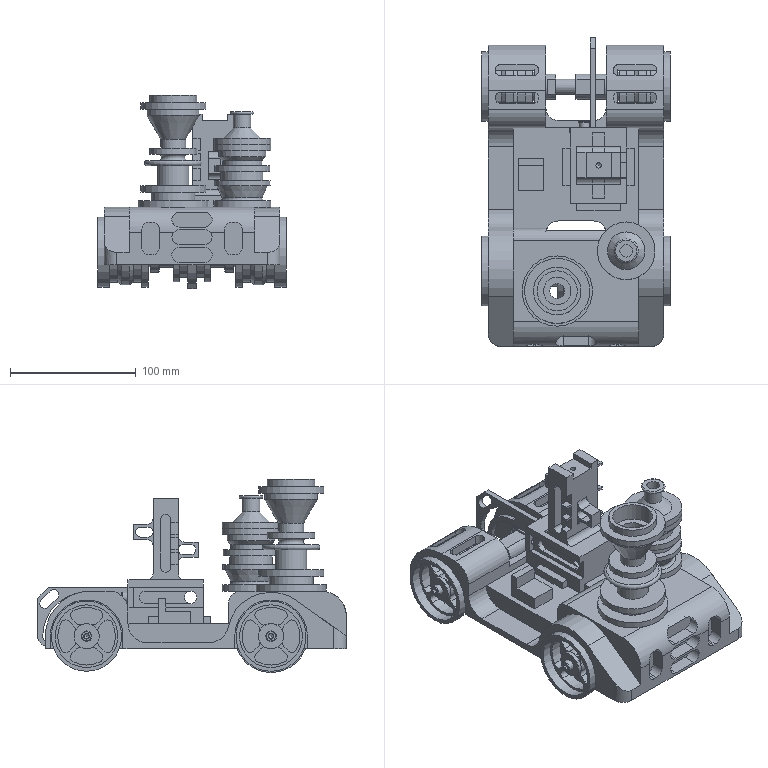Assembly | NX | mm | 29 component files | 81 solids | 972 faces | box 150 x 246 x 154 mm | volume 917936 mm3 | plane 477 | cylinder 340 | cone 83 | sphere 48 | torus 24 | commonest cylinder face diameters 8 x78 20 x49 46 x20 12 x18 28 x13 4.826 x12 16 x12 10 x10
Bill of materials:
GB-T70.1-2000,M5x10 | 6 |  | Hexagon Socket Head Cap Screw, GB-T 70.1-2000,M5x10
unnamed part 1 | 4 |  | Flat annular disc (washer-like ring) with a single concentric round through-hole; plain cylindrical outer edge.
unnamed part 2 | 1 |  | Symmetric stepped axisymmetric shaft with a central cluster of three raised flanges (tallest in the middle) flanked by stepped shoulders and long plain end journals; small axial hole at the shaft end.
unnamed part 3 | 4 |  | Spool- or rim-like axisymmetric hollow body: cylinder with raised end flanges and a raised central band with tapered edges; open end shows an inner hub with central bore connected to the rim by three curved spokes/webs.
GB-T276_60000-1994,61804 | 4 |  | Annular assembly that looks like an open radial ball bearing. It has a plain cylindrical outer ring, a concentric inner ring with a through bore, and a single row of spherical balls in the annular gap between the rings. No cage, shields or seals are visible.
unnamed part 4 | 1 |  | Axisymmetric flanged nozzle-like body: wide flat flange disc, a conical section rising to a narrow cylindrical neck with rounded bead lip at top, and a stepped cylindrical spigot below the flange; central through-bore.
unnamed part 5 | 3 |  | Plain thick-walled cylindrical tube/sleeve with a concentric through-bore and flat square ends.
unnamed part 6 | 1 |  | Stepped cylindrical shaft with several diameter changes, a narrow raised collar, a reduced neck in the middle, and flat milled faces on two of the larger sections; small axial hole at one end.
unnamed part 7 | 1 |  | Prismatic block-type body: rectangular base with side grooves/steps and a long slot, supporting a narrower vertical column with a top notch, a small top hole, side lugs with obround slots, and a row of thin horizontal fins/ribs along one side.
unnamed part 8 | 1 |  | Axisymmetric stacked-flange body: several disc flanges separated by necks, a large cup/counterbore at the top, a flared conical section with filleted root near the bottom, and a small cylindrical pin projecting from the bottom.
unnamed part 9 | 1 |  | Plate-like saddle/clamp body with two parallel half-round arched channels across its width, a flat central deck with small raised blocks and ribs, several obround slots in the arches and end wall, a large round hole with a flat (D-shaped) and small holes.
unnamed part 10 | 1 |  | Axisymmetric multi-stage body with a central through-bore: top cylindrical rim with flange, a converging funnel cone, narrow neck, a flange and rounded bead ring separated by a filleted groove, a cylindrical stem, and two lower flanges with a short bottom spigot.
unnamed part 11 | 1 |  | L-shaped flat bracket of uniform thickness: short leg with an obround slot, long arm ending in a curved hook-like lobe containing a long arcuate slot and an angled obround slot, with a chamfered corner.
Mates:
1. fix | car_body 1 component
2. concentric | support_block 1 arc | car_body 1 edge
3. concentric | lamp_body 1 edge | car_body 1 edge
4. concentric | lamp_socket 1 edge | lamp_body 1 edge
5. concentric | column 1 edge | car_body 1 edge
6. touch align | rear_axle 1 face | car_body 1 face
7. center | rear_axle 1 face | rear_axle 1 face | car_body 1 face | car_body 1 face
8. touch align | front_axle 1 face | car_body 1 face
9. center | front_axle 1 face | front_axle 1 face | car_body 1 face | car_body 1 face
10. concentric | GB-T276_60000-1994_61804 4 edge | car_body 1 edge
11. bond | car_body 1 component | assembly component
12. bond | GB-T276_60000-1994_61804 4 component | assembly component
13. bond | GB-T276_60000-1994_61804 3 component | assembly component
14. linear | assembly datumaxis | assembly cartesiancoordinatesystem | assembly cartesiancoordinatesystem
15. concentric | spacer 2 edge | GB-T276_60000-1994_61804 3 edge
16. bond | car_body 1 component | assembly component
17. bond | spacer 3 component | assembly component
18. bond | spacer 1 component | assembly component
19. linear | assembly datumaxis | assembly cartesiancoordinatesystem | assembly cartesiancoordinatesystem
20. concentric | wheel 4 edge | rear_axle 1 edge
21. concentric | wheel 3 edge | spacer 1 edge
22. bond | wheel 4 component | assembly component
23. bond | wheel 2 component | assembly component
24. linear | assembly datumaxis | assembly cartesiancoordinatesystem | assembly cartesiancoordinatesystem
25. bond | wheel 3 component | assembly component
26. bond | wheel 1 component | assembly component
27. linear | assembly datumaxis | assembly cartesiancoordinatesystem | assembly cartesiancoordinatesystem
28. concentric | circlip 4 edge | wheel 4 edge
29. concentric | circlip 3 edge | wheel 3 edge
30. bond | circlip 3 component | assembly component
31. bond | circlip 2 component | assembly component
32. linear | assembly datumaxis | assembly cartesiancoordinatesystem | assembly cartesiancoordinatesystem
33. bond | circlip 4 component | assembly component
34. bond | circlip 1 component | assembly component
35. linear | assembly datumaxis | assembly cartesiancoordinatesystem | assembly cartesiancoordinatesystem
36. concentric | GB-T70_1-2000_M5x10 6 edge | circlip 4 edge
37. bond | GB-T70_1-2000_M5x10 5 component | assembly component
38. bond | GB-T70_1-2000_M5x10 4 component | assembly component
39. linear | assembly datumaxis | assembly cartesiancoordinatesystem | assembly cartesiancoordinatesystem
40. bond | GB-T70_1-2000_M5x10 6 component | assembly component
41. bond | GB-T70_1-2000_M5x10 3 component | assembly component
42. linear | assembly datumaxis | assembly cartesiancoordinatesystem | assembly cartesiancoordinatesystem
43. concentric | GB-T276_60000-1994_61804 2 edge | car_body 1 edge
44. bond | GB-T276_60000-1994_61804 2 component | assembly component
45. bond | GB-T276_60000-1994_61804 1 component | assembly component
46. linear | assembly datumaxis | assembly cartesiancoordinatesystem | assembly cartesiancoordinatesystem
47. concentric | bracket 1 edge | support_block 1 arc